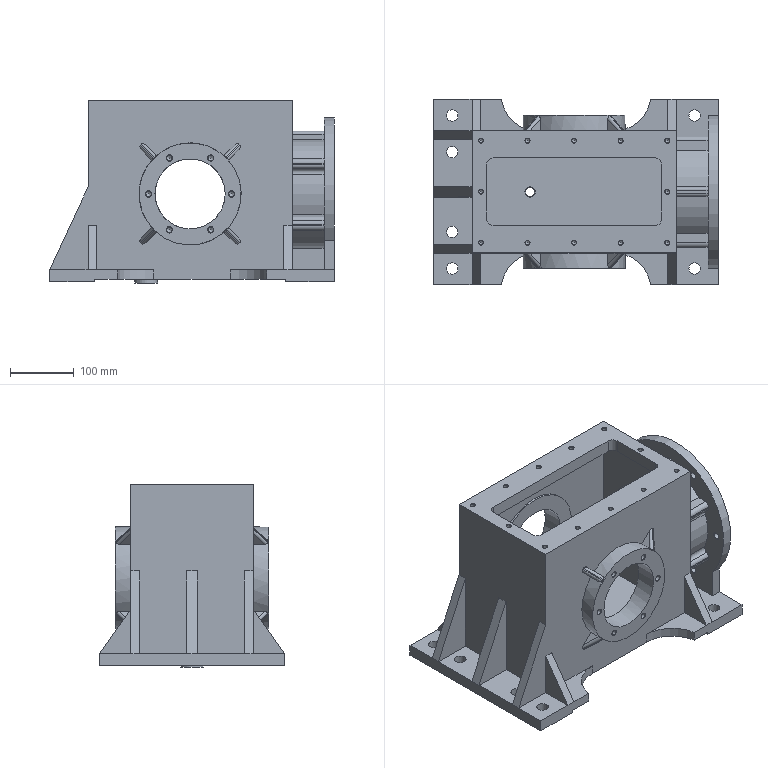Component | NX | HOUSING_SHELL | 1 solid | 252 faces | volume 5180559 mm3 | plane 98 | cylinder 92 | cone 62 | commonest cylinder face diameters 8 x16 14 x13 6.8 x12 8.5 x12 18 x8 170 x6 10.3 x6 160 x4